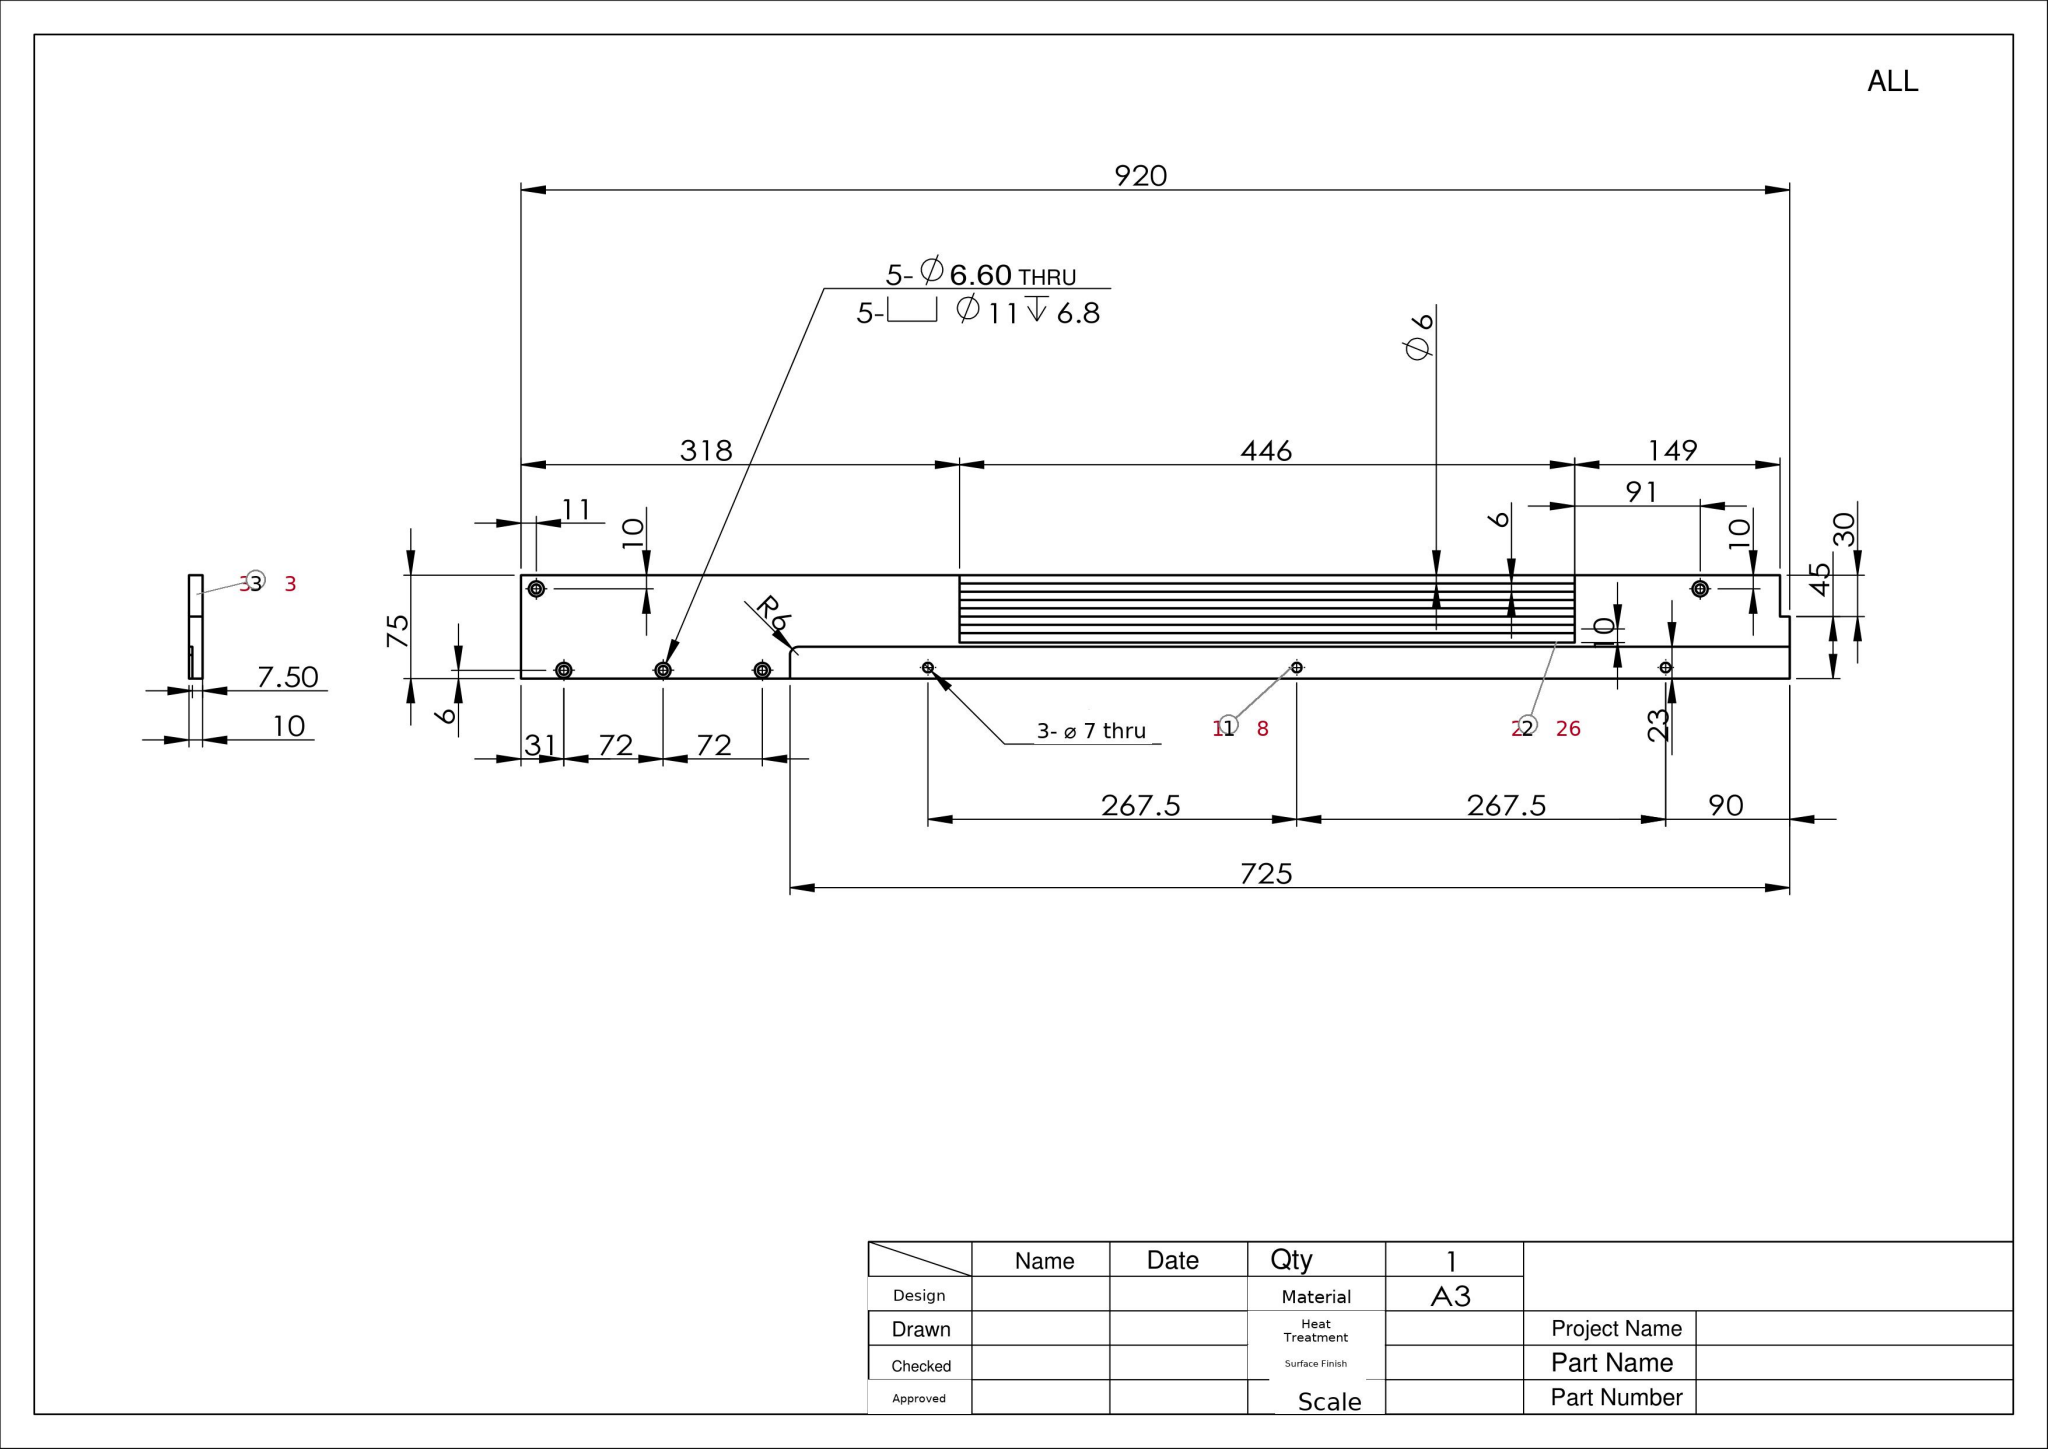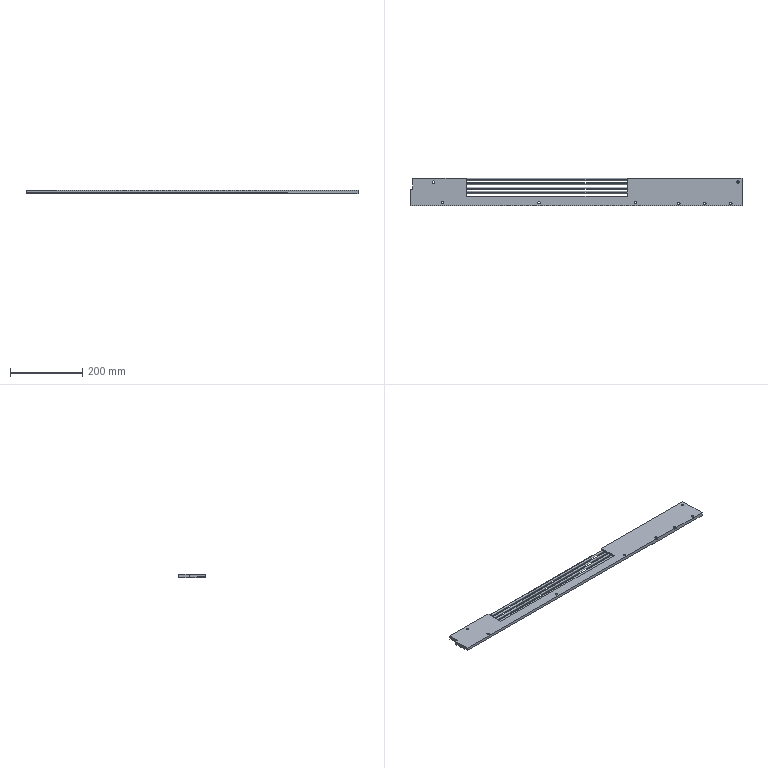Part | SolidWorks | mm | 1 solid | 57 faces | box 920 x 75 x 10 mm | volume 473489 mm3 | cylinder 35 | plane 22 | commonest cylinder face diameters 6.6 x10 11 x10 6 x8 7 x6 12 x1
build123d program:
from build123d import *

# Parameters (mm, degrees)
SKETCH1_W                                            = 1020
SKETCH1_H                                            = 75
EXTRUDE1_DEPTH                                       = 10
SKETCH2_W                                            = 377.249
SKETCH2_H                                            = 184.95
CUT_EXTRUDE1_DEPTH                                   = 1023.803
SKETCH3_W                                            = 446
SKETCH3_H                                            = 197.561
CUT_EXTRUDE2_DEPTH                                   = 1023.803
SKETCH4_R                                            = 3
EXTRUDE2_DEPTH                                       = 446
SKETCH5_W                                            = 1001.916
SKETCH5_H                                            = 184.536
CUT_EXTRUDE3_DEPTH                                   = 2.5
FILLET1_R                                            = 6
SKETCH6_R                                            = 3.5
CUT_EXTRUDE4_DEPTH                                   = 1023.781
HOLE_SIZE_ACCORDING_TO_HEXAGON_SOCKET_HE_D           = 6.6
HOLE_SIZE_ACCORDING_TO_HEXAGON_SOCKET_HE_CBORE_D     = 11
HOLE_SIZE_ACCORDING_TO_HEXAGON_SOCKET_HE_CBORE_DEPTH = 6.8
SKETCH9_W                                            = 201.394
SKETCH9_H                                            = 241.293
CUT_EXTRUDE5_DEPTH                                   = 1023.803
SKETCH10_W                                           = 10
SKETCH10_H                                           = 30
EXTRUDE3_DEPTH                                       = 3


with BuildPart() as part:
    # Sketch1 → Extrude1 (new body)
    with BuildSketch(Plane.XY):
        with Locations((510, 37.5)):
            Rectangle(SKETCH1_W, SKETCH1_H)
    extrude(amount=EXTRUDE1_DEPTH)

    # Sketch2 → Cut-Extrude1 (cut, through all)
    with BuildSketch(Plane.XY.offset(10)):
        with Locations((-78.625, 137.475)):
            Rectangle(SKETCH2_W, SKETCH2_H)
    extrude(amount=-CUT_EXTRUDE1_DEPTH, mode=Mode.SUBTRACT)

    # Sketch3 → Cut-Extrude2 (cut, through all)
    with BuildSketch(Plane(origin=(0, 0, 0), x_dir=(-1, 0, 0), z_dir=(0, 0, -1))):
        with Locations((-479, 124.781)):
            Rectangle(SKETCH3_W, SKETCH3_H)
    extrude(amount=-CUT_EXTRUDE2_DEPTH, mode=Mode.SUBTRACT)

    # Sketch4 → Extrude2 (add)
    with BuildSketch(Plane(origin=(256, 0, 0), x_dir=(0, 0, -1), z_dir=(1, 0, 0))):
        with Locations(Location((-3, 72, 0), (0, 0, 90))):
            Circle(SKETCH4_R)
        with Locations((-3, 60)):
            Circle(SKETCH4_R)
        with Locations((-3, 36)):
            Circle(SKETCH4_R)
        with Locations((-3, 48)):
            Circle(SKETCH4_R)
    extrude(amount=EXTRUDE2_DEPTH)

    # Sketch5 → Cut-Extrude3 (cut)
    with BuildSketch(Plane(origin=(0, 0, 0), x_dir=(-1, 0, 0), z_dir=(0, 0, -1))):
        with Locations((-324.042, -69.268)):
            Rectangle(SKETCH5_W, SKETCH5_H)
    extrude(amount=-CUT_EXTRUDE3_DEPTH, mode=Mode.SUBTRACT)

    # Fillet1
    fillet1_edges = [part.edges().sort_by_distance(p)[0] for p in [
        (825, 23, 1.25),
    ]]
    fillet(fillet1_edges, radius=FILLET1_R)

    # Sketch6 → Cut-Extrude4 (cut, through all)
    with BuildSketch(Plane(origin=(0, 0, 2.5), x_dir=(-1, 0, 0), z_dir=(0, 0, -1))):
        with Locations((-725, 8)):
            Circle(SKETCH6_R)
        with Locations((-457.5, 8)):
            Circle(SKETCH6_R)
        with Locations((-190, 8)):
            Circle(SKETCH6_R)
    extrude(amount=-CUT_EXTRUDE4_DEPTH, mode=Mode.SUBTRACT)

    # Hole Size according to Hexagon Socket He (through all)
    with Locations(Plane(origin=(1009, 65, 0), x_dir=(-1, 0, 0), z_dir=(0, 0, -1))):
        with Locations((0, 0), (92, -59), (20, -59), (164, -59), (844, 0)):
            CounterBoreHole(HOLE_SIZE_ACCORDING_TO_HEXAGON_SOCKET_HE_D / 2, HOLE_SIZE_ACCORDING_TO_HEXAGON_SOCKET_HE_CBORE_D / 2, HOLE_SIZE_ACCORDING_TO_HEXAGON_SOCKET_HE_CBORE_DEPTH)

    # Sketch9 → Cut-Extrude5 (cut, through all)
    with BuildSketch(Plane(origin=(0, 0, 0), x_dir=(-1, 0, 0), z_dir=(0, 0, -1))):
        with Locations((0.6972, 11.778)):
            Rectangle(SKETCH9_W, SKETCH9_H)
    extrude(amount=-CUT_EXTRUDE5_DEPTH, mode=Mode.SUBTRACT)

    # Sketch10 → Extrude3 (add)
    with BuildSketch(Plane.ZY.offset(-110)):
        with Locations((5, 60)):
            Rectangle(SKETCH10_W, SKETCH10_H)
    extrude(amount=EXTRUDE3_DEPTH)


solid = part.part